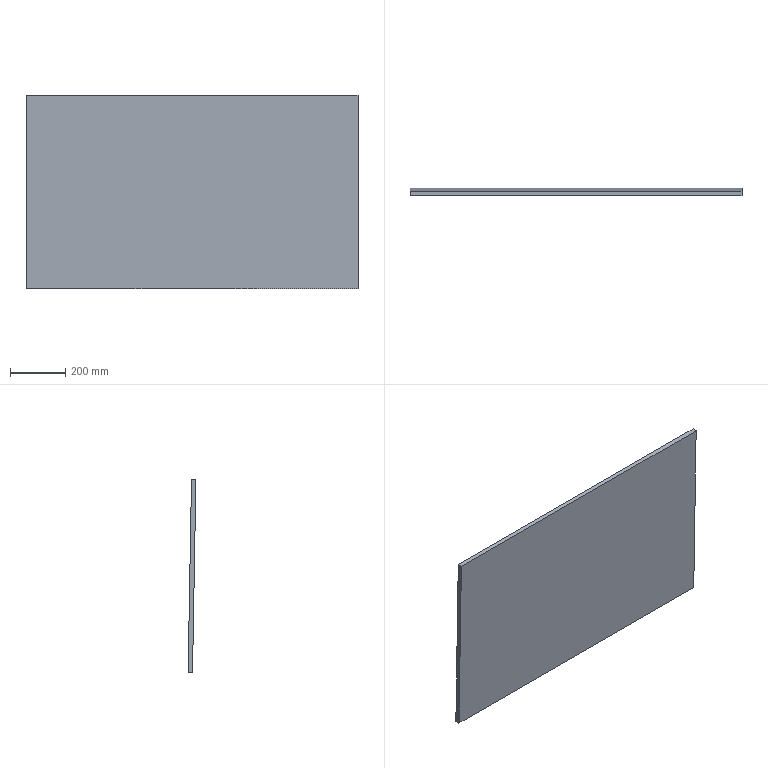Component | SolidWorks | EdgeTrimmingTableSLDPRT-1 | 1 solid | 6 faces | box 1200 x 28.21 x 700.17 mm | volume 13440000 mm3 | plane 6 | material Plain Carbon Steel
build123d program:
from build123d import *

# Parameters (mm, degrees)
SKETCH1_W      = 1200
SKETCH1_H      = 700
EXTRUDE1_DEPTH = 16


with BuildPart() as part:
    # Sketch1 → Extrude1 (new body)
    with BuildSketch(Plane.XY):
        Rectangle(SKETCH1_W, SKETCH1_H)
    extrude(amount=EXTRUDE1_DEPTH)


solid = part.part

# Placed as in the assembly
solid = solid.moved(Location((277.004, 1181.906, 560.041), (91, 0, 0)))
STEP:
#1=COLOUR_RGB('',0.7922,0.8196,0.9333);
#2=FILL_AREA_STYLE_COLOUR('',#1);
#3=FILL_AREA_STYLE('',(#2));
#4=SURFACE_STYLE_FILL_AREA(#3);
#5=SURFACE_SIDE_STYLE('',(#4));
#6=SURFACE_STYLE_USAGE(.BOTH.,#5);
#7=PRESENTATION_STYLE_ASSIGNMENT((#6));
#8=CARTESIAN_POINT('',(34.528,45.661,35.815));
#9=VERTEX_POINT('',#8);
#10=CARTESIAN_POINT('',(34.528,46.142,8.26));
#11=VERTEX_POINT('',#10);
#12=CARTESIAN_POINT('',(34.528,46.142,8.26));
#13=DIRECTION('',(-0.,0.01745,-0.9998));
#14=VECTOR('',#13,39.37);
#15=LINE('',#12,#14);
#16=EDGE_CURVE('',#9,#11,#15,.T.);
#17=ORIENTED_EDGE('',*,*,#16,.T.);
#18=CARTESIAN_POINT('',(34.528,46.772,8.271));
#19=VERTEX_POINT('',#18);
#20=CARTESIAN_POINT('',(34.528,46.772,8.271));
#21=DIRECTION('',(0.,-0.9998,-0.01745));
#22=VECTOR('',#21,39.37);
#23=LINE('',#20,#22);
#24=EDGE_CURVE('',#19,#11,#23,.T.);
#25=ORIENTED_EDGE('',*,*,#24,.F.);
#26=CARTESIAN_POINT('',(34.528,46.291,35.826));
#27=VERTEX_POINT('',#26);
#28=CARTESIAN_POINT('',(34.528,46.772,8.271));
#29=DIRECTION('',(-0.,0.01745,-0.9998));
#30=VECTOR('',#29,39.37);
#31=LINE('',#28,#30);
#32=EDGE_CURVE('',#27,#19,#31,.T.);
#33=ORIENTED_EDGE('',*,*,#32,.F.);
#34=CARTESIAN_POINT('',(34.528,46.291,35.826));
#35=DIRECTION('',(0.,-0.9998,-0.01745));
#36=VECTOR('',#35,39.37);
#37=LINE('',#34,#36);
#38=EDGE_CURVE('',#27,#9,#37,.T.);
#39=ORIENTED_EDGE('',*,*,#38,.T.);
#40=EDGE_LOOP('',(#17,#25,#33,#39));
#41=FACE_OUTER_BOUND('',#40,.T.);
#42=CARTESIAN_POINT('',(34.528,46.772,8.271));
#43=DIRECTION('',(-1.,-0.,-0.));
#44=DIRECTION('',(0.,-0.01745,0.9998));
#45=AXIS2_PLACEMENT_3D('',#42,#43,#44);
#46=PLANE('',#45);
#47=ADVANCED_FACE('',(#41),#46,.F.);
#48=CARTESIAN_POINT('',(-12.716,46.142,8.26));
#49=VERTEX_POINT('',#48);
#50=CARTESIAN_POINT('',(-12.716,46.142,8.26));
#51=DIRECTION('',(-1.,-0.,-0.));
#52=VECTOR('',#51,39.37);
#53=LINE('',#50,#52);
#54=EDGE_CURVE('',#11,#49,#53,.T.);
#55=ORIENTED_EDGE('',*,*,#54,.T.);
#56=CARTESIAN_POINT('',(-12.716,46.772,8.271));
#57=VERTEX_POINT('',#56);
#58=CARTESIAN_POINT('',(-12.716,46.772,8.271));
#59=DIRECTION('',(0.,-0.9998,-0.01745));
#60=VECTOR('',#59,39.37);
#61=LINE('',#58,#60);
#62=EDGE_CURVE('',#57,#49,#61,.T.);
#63=ORIENTED_EDGE('',*,*,#62,.F.);
#64=CARTESIAN_POINT('',(-12.716,46.772,8.271));
#65=DIRECTION('',(-1.,-0.,-0.));
#66=VECTOR('',#65,39.37);
#67=LINE('',#64,#66);
#68=EDGE_CURVE('',#19,#57,#67,.T.);
#69=ORIENTED_EDGE('',*,*,#68,.F.);
#70=ORIENTED_EDGE('',*,*,#24,.T.);
#71=EDGE_LOOP('',(#55,#63,#69,#70));
#72=FACE_OUTER_BOUND('',#71,.T.);
#73=CARTESIAN_POINT('',(-12.716,46.772,8.271));
#74=DIRECTION('',(-0.,-0.01745,0.9998));
#75=DIRECTION('',(0.,-0.9998,-0.01745));
#76=AXIS2_PLACEMENT_3D('',#73,#74,#75);
#77=PLANE('',#76);
#78=ADVANCED_FACE('',(#72),#77,.F.);
#79=CARTESIAN_POINT('',(-12.716,45.661,35.815));
#80=VERTEX_POINT('',#79);
#81=CARTESIAN_POINT('',(-12.716,46.142,8.26));
#82=DIRECTION('',(0.,-0.01745,0.9998));
#83=VECTOR('',#82,39.37);
#84=LINE('',#81,#83);
#85=EDGE_CURVE('',#49,#80,#84,.T.);
#86=ORIENTED_EDGE('',*,*,#85,.T.);
#87=CARTESIAN_POINT('',(-12.716,46.291,35.826));
#88=VERTEX_POINT('',#87);
#89=CARTESIAN_POINT('',(-12.716,46.291,35.826));
#90=DIRECTION('',(0.,-0.9998,-0.01745));
#91=VECTOR('',#90,39.37);
#92=LINE('',#89,#91);
#93=EDGE_CURVE('',#88,#80,#92,.T.);
#94=ORIENTED_EDGE('',*,*,#93,.F.);
#95=CARTESIAN_POINT('',(-12.716,46.772,8.271));
#96=DIRECTION('',(0.,-0.01745,0.9998));
#97=VECTOR('',#96,39.37);
#98=LINE('',#95,#97);
#99=EDGE_CURVE('',#57,#88,#98,.T.);
#100=ORIENTED_EDGE('',*,*,#99,.F.);
#101=ORIENTED_EDGE('',*,*,#62,.T.);
#102=EDGE_LOOP('',(#86,#94,#100,#101));
#103=FACE_OUTER_BOUND('',#102,.T.);
#104=CARTESIAN_POINT('',(-12.716,46.772,8.271));
#105=DIRECTION('',(1.,0.,-0.));
#106=DIRECTION('',(-0.,0.01745,-0.9998));
#107=AXIS2_PLACEMENT_3D('',#104,#105,#106);
#108=PLANE('',#107);
#109=ADVANCED_FACE('',(#103),#108,.F.);
#110=CARTESIAN_POINT('',(-12.716,45.661,35.815));
#111=DIRECTION('',(1.,0.,0.));
#112=VECTOR('',#111,39.37);
#113=LINE('',#110,#112);
#114=EDGE_CURVE('',#80,#9,#113,.T.);
#115=ORIENTED_EDGE('',*,*,#114,.T.);
#116=ORIENTED_EDGE('',*,*,#38,.F.);
#117=CARTESIAN_POINT('',(-12.716,46.291,35.826));
#118=DIRECTION('',(1.,0.,0.));
#119=VECTOR('',#118,39.37);
#120=LINE('',#117,#119);
#121=EDGE_CURVE('',#88,#27,#120,.T.);
#122=ORIENTED_EDGE('',*,*,#121,.F.);
#123=ORIENTED_EDGE('',*,*,#93,.T.);
#124=EDGE_LOOP('',(#115,#116,#122,#123));
#125=FACE_OUTER_BOUND('',#124,.T.);
#126=CARTESIAN_POINT('',(-12.716,46.291,35.826));
#127=DIRECTION('',(0.,0.01745,-0.9998));
#128=DIRECTION('',(-0.,0.9998,0.01745));
#129=AXIS2_PLACEMENT_3D('',#126,#127,#128);
#130=PLANE('',#129);
#131=ADVANCED_FACE('',(#125),#130,.F.);
#132=ORIENTED_EDGE('',*,*,#32,.T.);
#133=ORIENTED_EDGE('',*,*,#68,.T.);
#134=ORIENTED_EDGE('',*,*,#99,.T.);
#135=ORIENTED_EDGE('',*,*,#121,.T.);
#136=EDGE_LOOP('',(#132,#133,#134,#135));
#137=FACE_OUTER_BOUND('',#136,.T.);
#138=CARTESIAN_POINT('',(34.528,46.291,35.826));
#139=DIRECTION('',(-0.,0.9998,0.01745));
#140=DIRECTION('',(1.,0.,0.));
#141=AXIS2_PLACEMENT_3D('',#138,#139,#140);
#142=PLANE('',#141);
#143=ADVANCED_FACE('',(#137),#142,.T.);
#144=ORIENTED_EDGE('',*,*,#16,.F.);
#145=ORIENTED_EDGE('',*,*,#114,.F.);
#146=ORIENTED_EDGE('',*,*,#85,.F.);
#147=ORIENTED_EDGE('',*,*,#54,.F.);
#148=EDGE_LOOP('',(#144,#145,#146,#147));
#149=FACE_OUTER_BOUND('',#148,.T.);
#150=CARTESIAN_POINT('',(34.528,45.661,35.815));
#151=DIRECTION('',(-0.,0.9998,0.01745));
#152=DIRECTION('',(1.,0.,0.));
#153=AXIS2_PLACEMENT_3D('',#150,#151,#152);
#154=PLANE('',#153);
#155=ADVANCED_FACE('',(#149),#154,.F.);
#156=CLOSED_SHELL('',(#47,#78,#109,#131,#143,#155));
#157=MANIFOLD_SOLID_BREP('',#156);
#158=STYLED_ITEM('',(#7),#157);
#159=(LENGTH_UNIT()NAMED_UNIT(*)SI_UNIT($,.METRE.));
#160=LENGTH_MEASURE_WITH_UNIT(LENGTH_MEASURE(0.0254),#159);
#161=DIMENSIONAL_EXPONENTS(1.,0.,0.,0.,0.,0.,0.);
#162=(CONVERSION_BASED_UNIT('',#160)LENGTH_UNIT()NAMED_UNIT(#161));
#163=UNCERTAINTY_MEASURE_WITH_UNIT(LENGTH_MEASURE(0.00001),#162,'','');
#164=(NAMED_UNIT(*)PLANE_ANGLE_UNIT()SI_UNIT($,.RADIAN.));
#165=(NAMED_UNIT(*)SI_UNIT($,.STERADIAN.)SOLID_ANGLE_UNIT());
#166=(GEOMETRIC_REPRESENTATION_CONTEXT(3)GLOBAL_UNCERTAINTY_ASSIGNED_CONTEXT((#163))GLOBAL_UNIT_ASSIGNED_CONTEXT((#162,#164,#165))REPRESENTATION_CONTEXT('',''));
#167=MECHANICAL_DESIGN_GEOMETRIC_PRESENTATION_REPRESENTATION('',(#158),#166);
#168=PRESENTATION_LAYER_ASSIGNMENT('','',(#158));
#169=CARTESIAN_POINT('',(0.,0.,0.));
#170=DIRECTION('',(0.,0.,1.));
#171=DIRECTION('',(1.,0.,0.));
#172=AXIS2_PLACEMENT_3D('',#169,#170,#171);
#173=(LENGTH_UNIT()NAMED_UNIT(*)SI_UNIT($,.METRE.));
#174=LENGTH_MEASURE_WITH_UNIT(LENGTH_MEASURE(0.0254),#173);
#175=DIMENSIONAL_EXPONENTS(1.,0.,0.,0.,0.,0.,0.);
#176=(CONVERSION_BASED_UNIT('',#174)LENGTH_UNIT()NAMED_UNIT(#175));
#177=UNCERTAINTY_MEASURE_WITH_UNIT(LENGTH_MEASURE(0.00001),#176,'','');
#178=(NAMED_UNIT(*)PLANE_ANGLE_UNIT()SI_UNIT($,.RADIAN.));
#179=(NAMED_UNIT(*)SI_UNIT($,.STERADIAN.)SOLID_ANGLE_UNIT());
#180=(GEOMETRIC_REPRESENTATION_CONTEXT(3)GLOBAL_UNCERTAINTY_ASSIGNED_CONTEXT((#177))GLOBAL_UNIT_ASSIGNED_CONTEXT((#176,#178,#179))REPRESENTATION_CONTEXT('',''));
#181=ADVANCED_BREP_SHAPE_REPRESENTATION('',(#157,#172),#180);